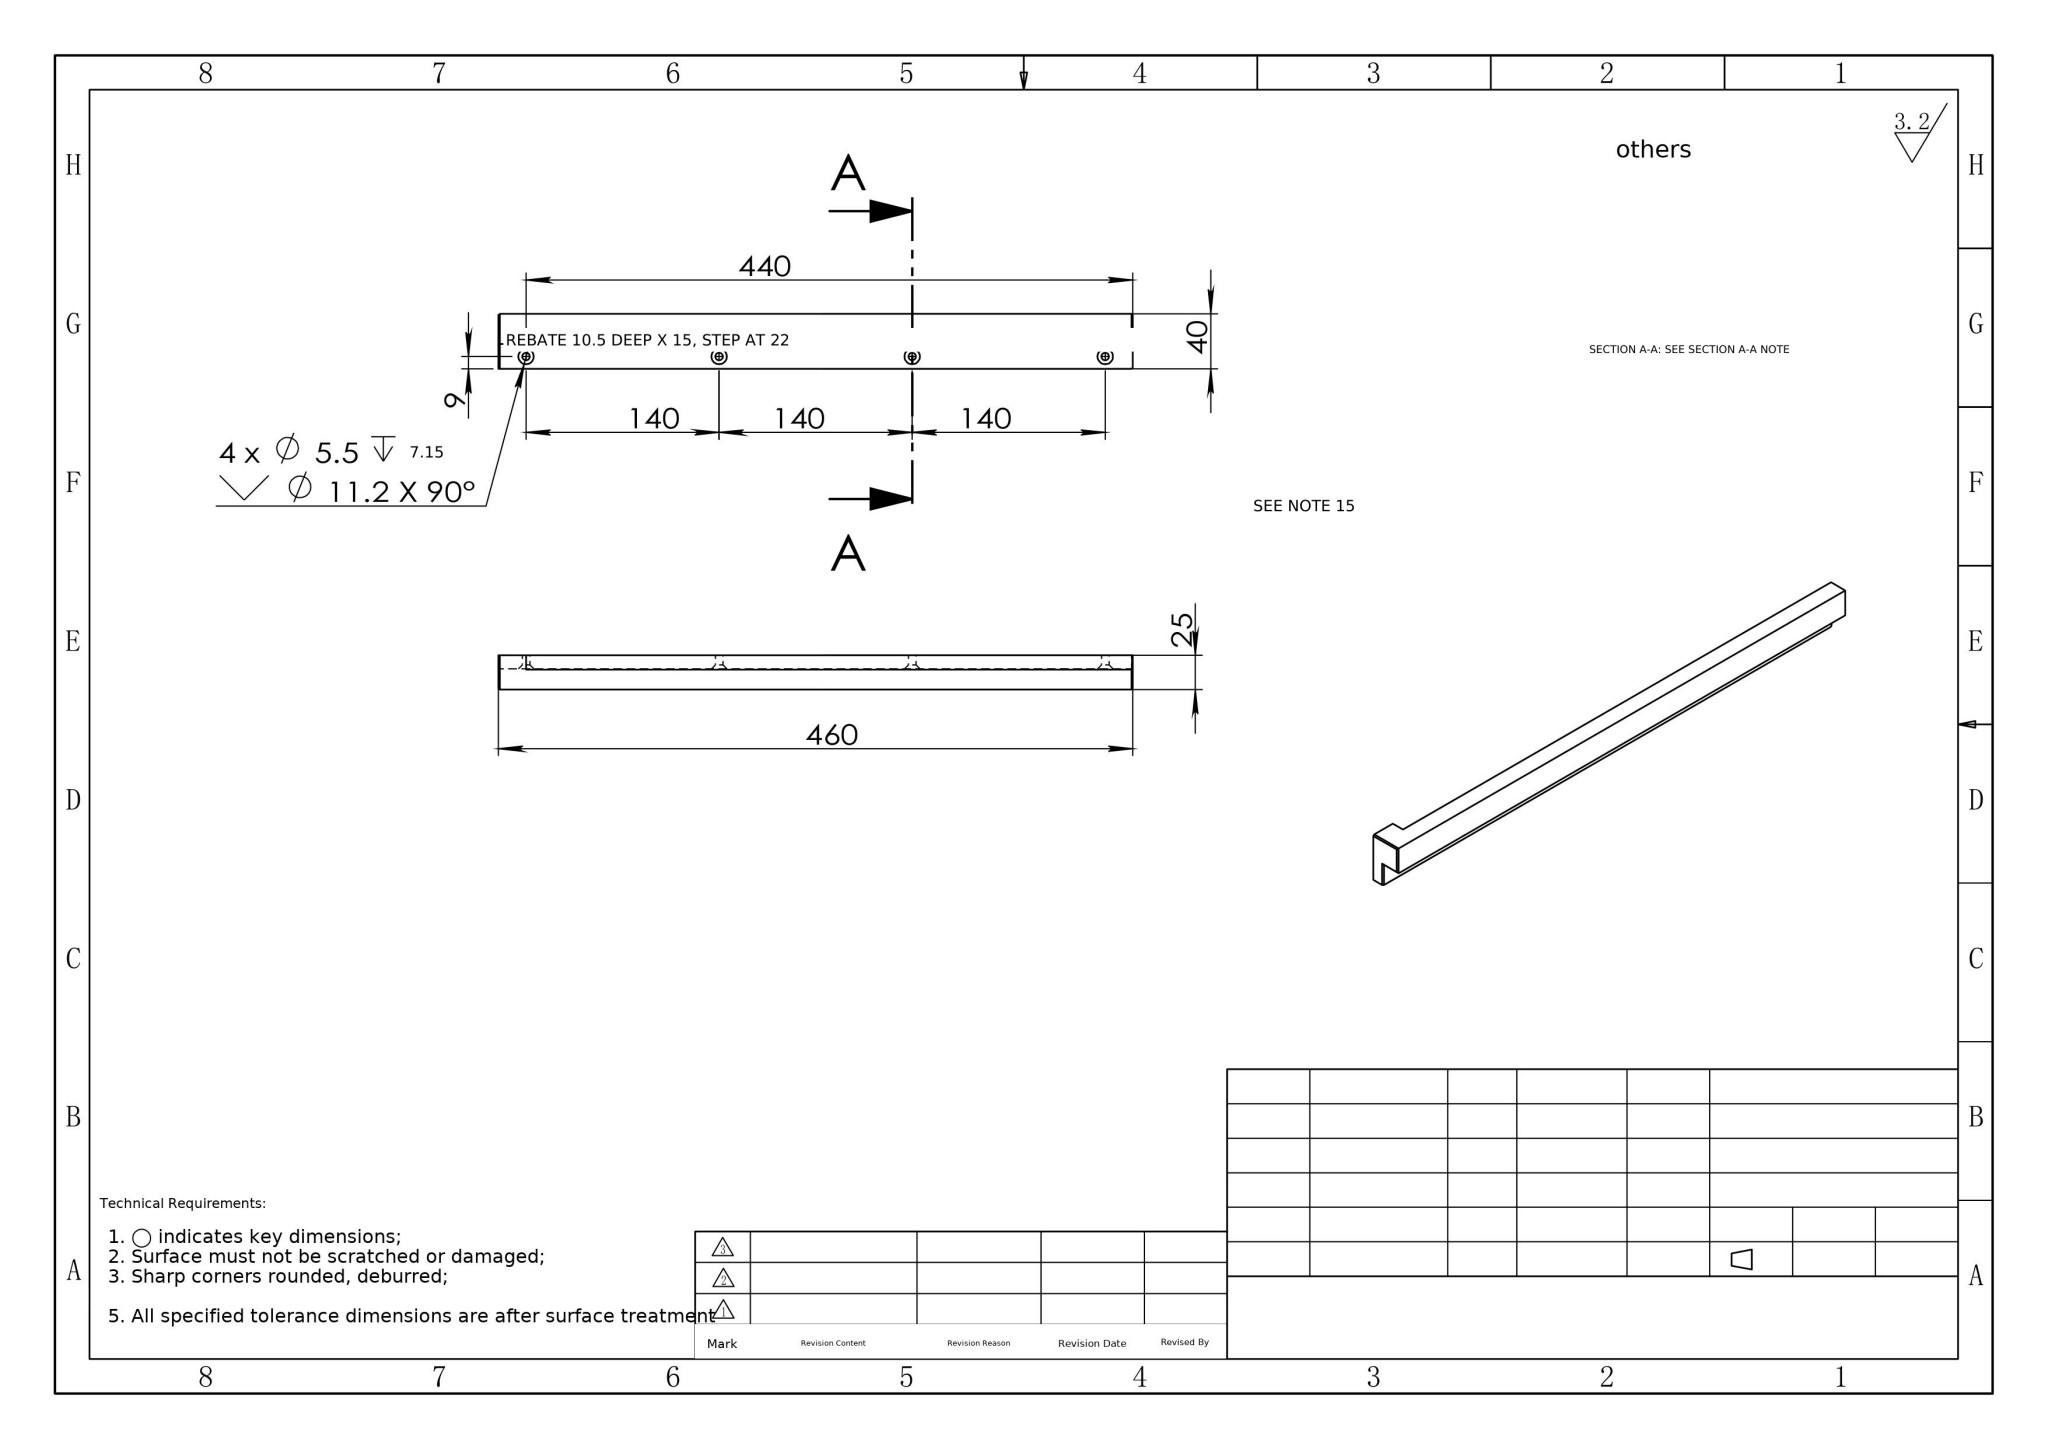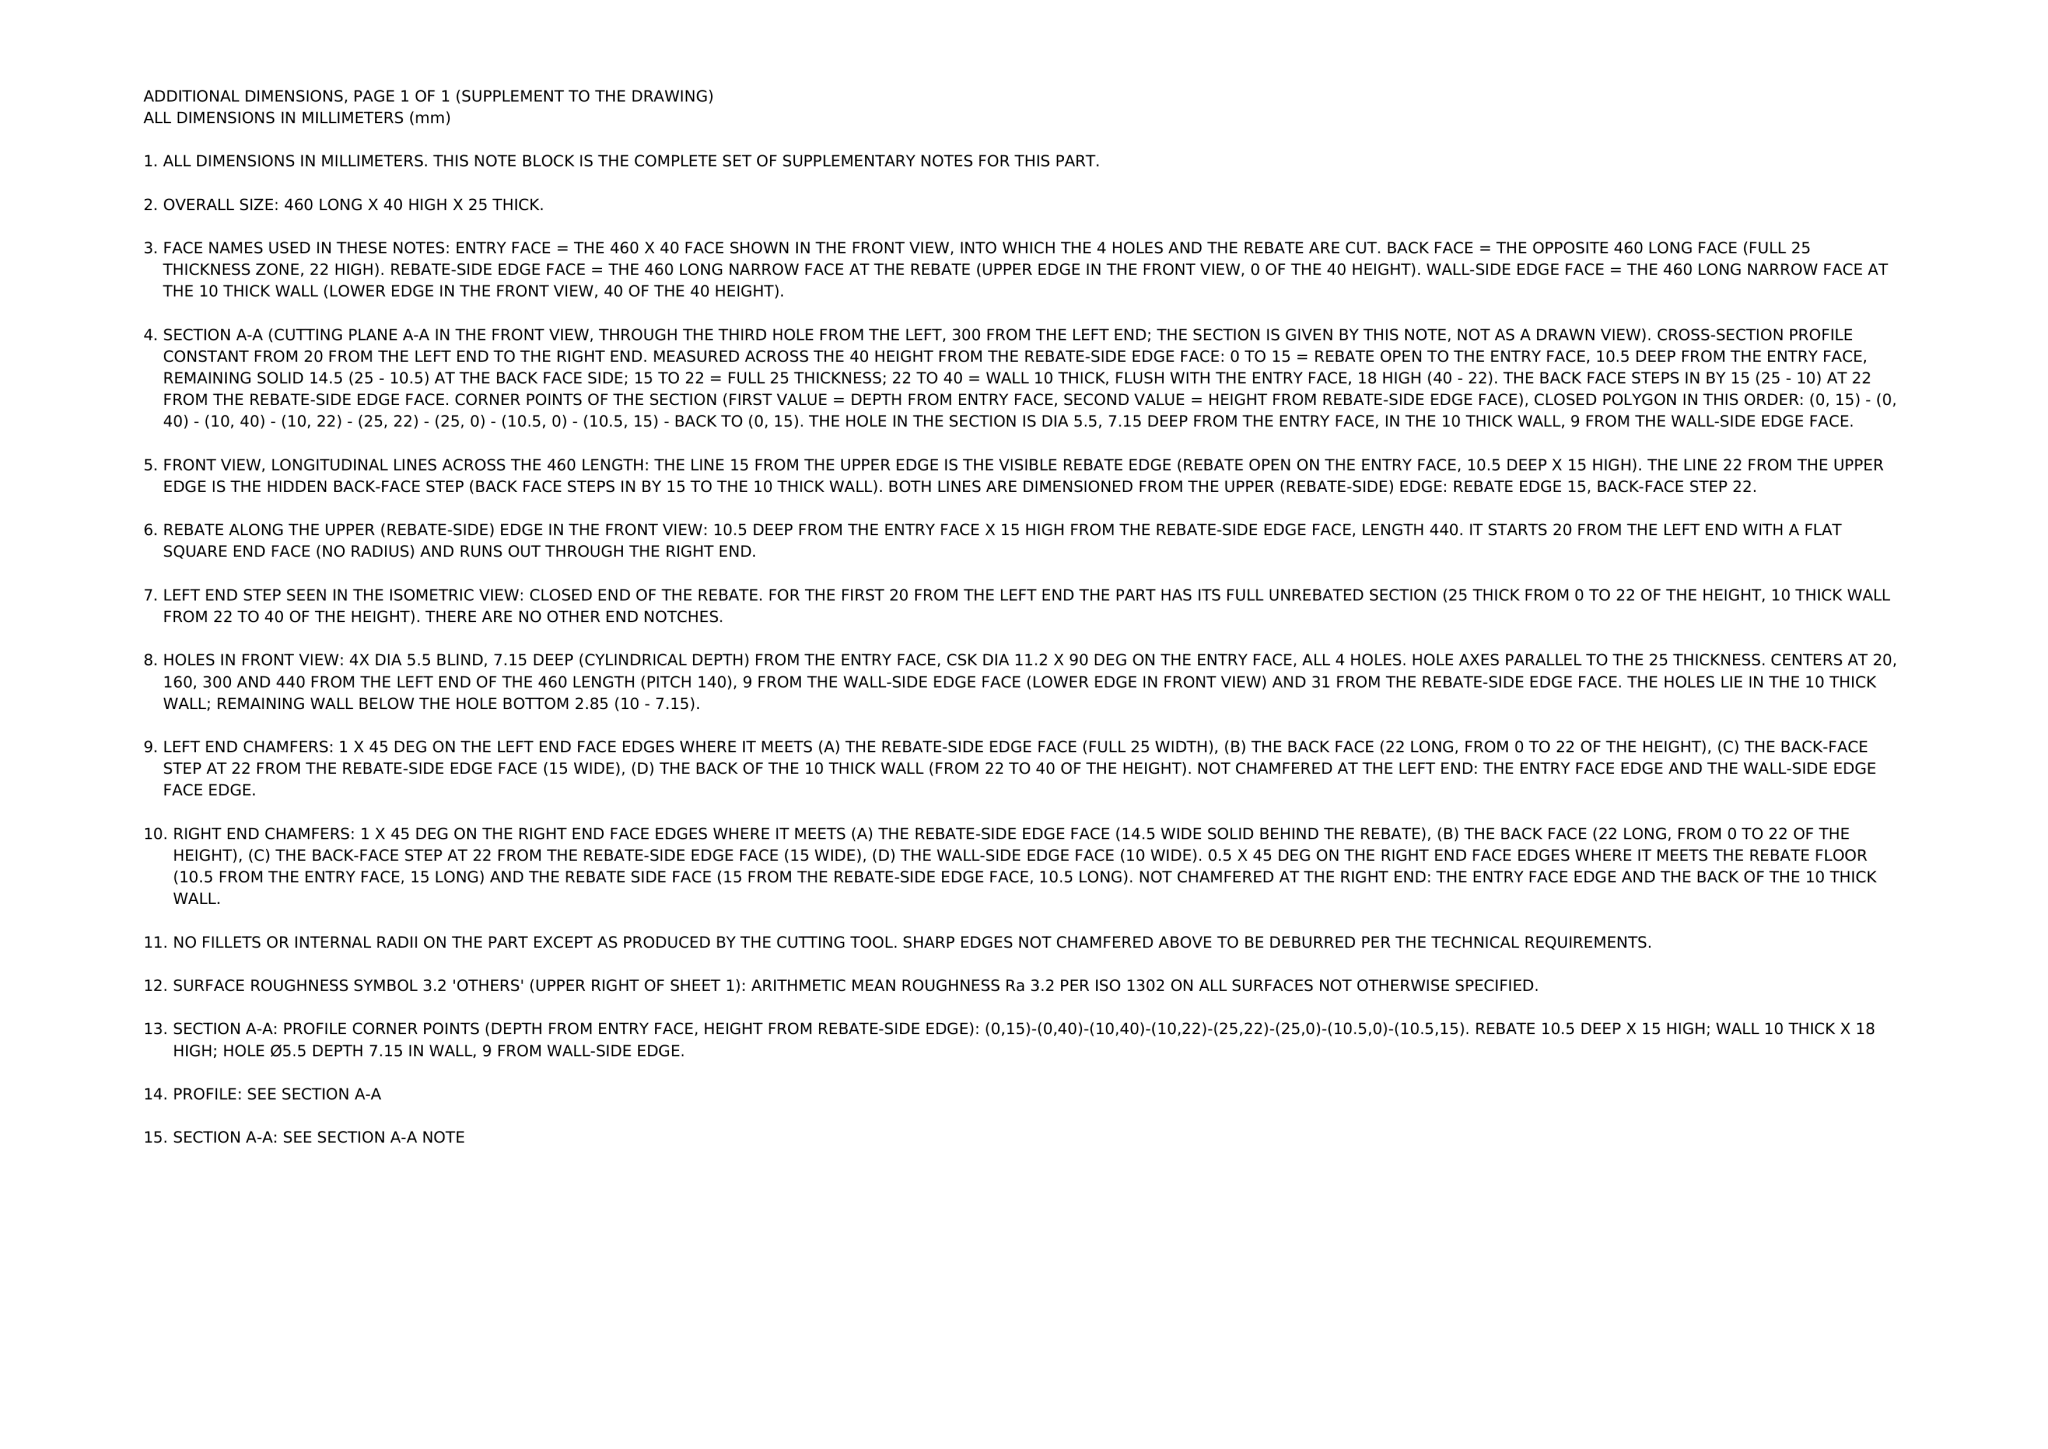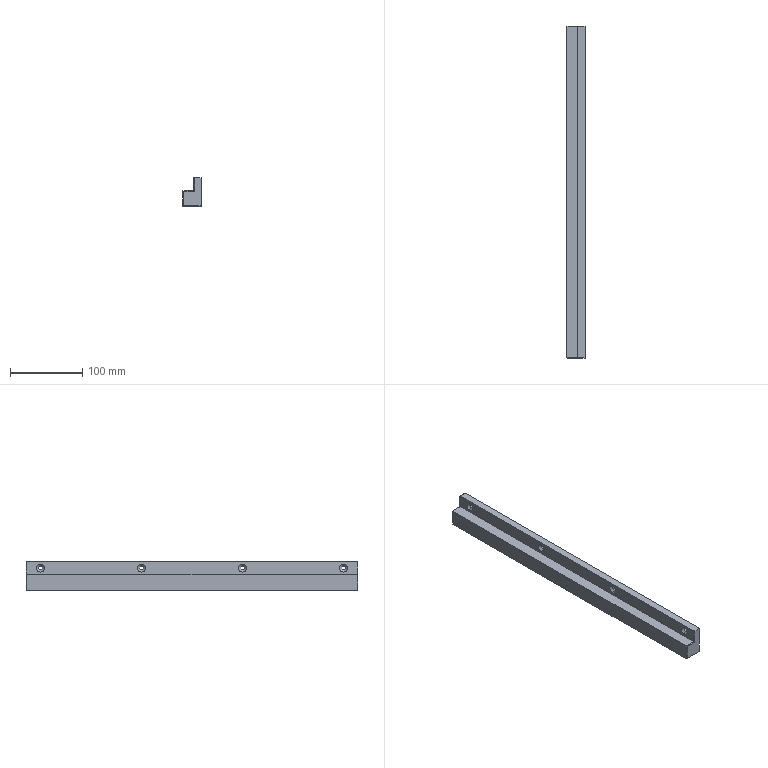Part | NX | mm | 1 solid | 37 faces | box 25 x 460 x 40 mm | volume 265099 mm3 | plane 21 | cone 8 | cylinder 8 | commonest cylinder face diameters 5.5 x8